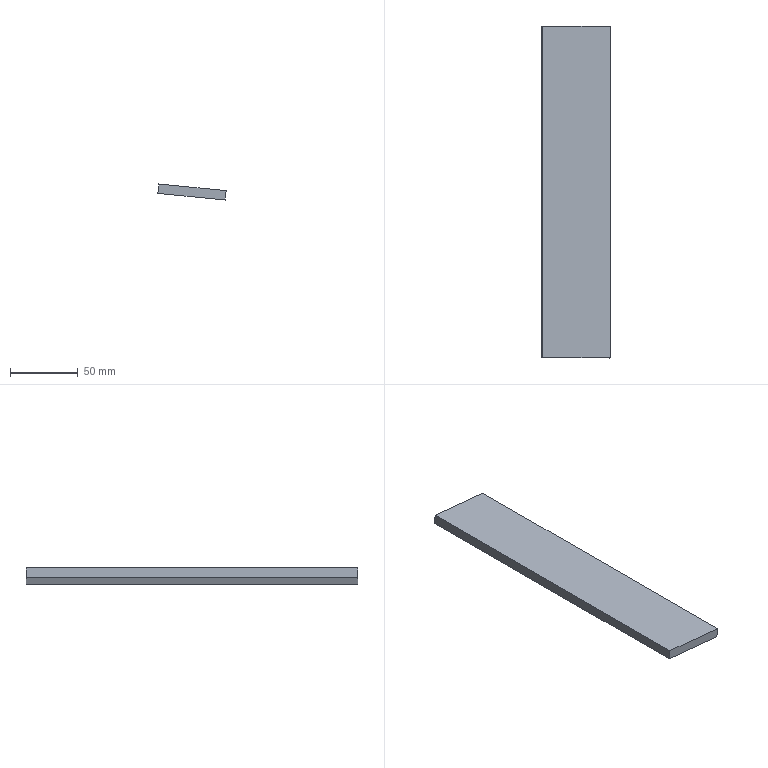Component | NX | MOVING_FRAME_BLOCK_3_2 | 1 solid | 6 faces | box 50.45 x 245 x 11.93 mm | volume 85750 mm3 | plane 6
STEP:
#1=CARTESIAN_POINT('',(0.,0.,0.));
#2=DIRECTION('',(0.,0.,1.));
#3=DIRECTION('',(1.,0.,0.));
#4=AXIS2_PLACEMENT_3D('',#1,#2,#3);
#5=CARTESIAN_POINT('',(470.025,-55.,468.347));
#6=VERTEX_POINT('',#5);
#7=CARTESIAN_POINT('',(469.329,-55.,461.382));
#8=VERTEX_POINT('',#7);
#9=CARTESIAN_POINT('',(470.025,-55.,468.347));
#10=DIRECTION('',(-0.09932,0.,-0.9951));
#11=VECTOR('',#10,1.);
#12=LINE('',#9,#11);
#13=CARTESIAN_POINT('',(470.025,190.,468.347));
#14=DIRECTION('',(-0.9951,0.,0.09932));
#15=DIRECTION('',(0.09932,0.,0.9951));
#16=AXIS2_PLACEMENT_3D('',#13,#14,#15);
#17=PLANE('',#16);
#18=CARTESIAN_POINT('',(0.,-245.));
#19=DIRECTION('',(-1.,0.));
#20=VECTOR('',#19,1.);
#21=LINE('',#18,#20);
#22=(GEOMETRIC_REPRESENTATION_CONTEXT(2)PARAMETRIC_REPRESENTATION_CONTEXT()REPRESENTATION_CONTEXT('',''));
#23=DEFINITIONAL_REPRESENTATION('',(#21),#22);
#24=PCURVE('',#17,#23);
#25=CARTESIAN_POINT('',(469.329,-55.,461.382));
#26=DIRECTION('',(0.,-1.,0.));
#27=DIRECTION('',(-0.09932,0.,-0.9951));
#28=AXIS2_PLACEMENT_3D('',#25,#26,#27);
#29=PLANE('',#28);
#30=CARTESIAN_POINT('',(-7.,-0.));
#31=DIRECTION('',(1.,0.));
#32=VECTOR('',#31,1.);
#33=LINE('',#30,#32);
#34=(GEOMETRIC_REPRESENTATION_CONTEXT(2)PARAMETRIC_REPRESENTATION_CONTEXT()REPRESENTATION_CONTEXT('',''));
#35=DEFINITIONAL_REPRESENTATION('',(#33),#34);
#36=PCURVE('',#29,#35);
#37=SURFACE_CURVE('',#12,(#24,#36),.PCURVE_S1.);
#38=EDGE_CURVE('',#6,#8,#37,.T.);
#39=ORIENTED_EDGE('',*,*,#38,.F.);
#40=CARTESIAN_POINT('',(470.025,190.,468.347));
#41=VERTEX_POINT('',#40);
#42=CARTESIAN_POINT('',(470.025,190.,468.347));
#43=DIRECTION('',(0.,-1.,0.));
#44=VECTOR('',#43,1.);
#45=LINE('',#42,#44);
#46=CARTESIAN_POINT('',(0.,0.));
#47=DIRECTION('',(0.,-1.));
#48=VECTOR('',#47,1.);
#49=LINE('',#46,#48);
#50=(GEOMETRIC_REPRESENTATION_CONTEXT(2)PARAMETRIC_REPRESENTATION_CONTEXT()REPRESENTATION_CONTEXT('',''));
#51=DEFINITIONAL_REPRESENTATION('',(#49),#50);
#52=PCURVE('',#17,#51);
#53=CARTESIAN_POINT('',(519.777,190.,463.381));
#54=DIRECTION('',(0.09932,0.,0.9951));
#55=DIRECTION('',(0.9951,0.,-0.09932));
#56=AXIS2_PLACEMENT_3D('',#53,#54,#55);
#57=PLANE('',#56);
#58=CARTESIAN_POINT('',(-50.,0.));
#59=DIRECTION('',(0.,-1.));
#60=VECTOR('',#59,1.);
#61=LINE('',#58,#60);
#62=(GEOMETRIC_REPRESENTATION_CONTEXT(2)PARAMETRIC_REPRESENTATION_CONTEXT()REPRESENTATION_CONTEXT('',''));
#63=DEFINITIONAL_REPRESENTATION('',(#61),#62);
#64=PCURVE('',#57,#63);
#65=SURFACE_CURVE('',#45,(#52,#64),.PCURVE_S1.);
#66=EDGE_CURVE('',#41,#6,#65,.T.);
#67=ORIENTED_EDGE('',*,*,#66,.F.);
#68=CARTESIAN_POINT('',(469.329,190.,461.382));
#69=VERTEX_POINT('',#68);
#70=CARTESIAN_POINT('',(470.025,190.,468.347));
#71=DIRECTION('',(-0.09932,0.,-0.9951));
#72=VECTOR('',#71,1.);
#73=LINE('',#70,#72);
#74=CARTESIAN_POINT('',(0.,0.));
#75=DIRECTION('',(-1.,0.));
#76=VECTOR('',#75,1.);
#77=LINE('',#74,#76);
#78=(GEOMETRIC_REPRESENTATION_CONTEXT(2)PARAMETRIC_REPRESENTATION_CONTEXT()REPRESENTATION_CONTEXT('',''));
#79=DEFINITIONAL_REPRESENTATION('',(#77),#78);
#80=PCURVE('',#17,#79);
#81=CARTESIAN_POINT('',(469.329,190.,461.382));
#82=DIRECTION('',(0.,-1.,0.));
#83=DIRECTION('',(-0.09932,0.,-0.9951));
#84=AXIS2_PLACEMENT_3D('',#81,#82,#83);
#85=PLANE('',#84);
#86=CARTESIAN_POINT('',(-7.,-0.));
#87=DIRECTION('',(1.,0.));
#88=VECTOR('',#87,1.);
#89=LINE('',#86,#88);
#90=(GEOMETRIC_REPRESENTATION_CONTEXT(2)PARAMETRIC_REPRESENTATION_CONTEXT()REPRESENTATION_CONTEXT('',''));
#91=DEFINITIONAL_REPRESENTATION('',(#89),#90);
#92=PCURVE('',#85,#91);
#93=SURFACE_CURVE('',#73,(#80,#92),.PCURVE_S1.);
#94=EDGE_CURVE('',#41,#69,#93,.T.);
#95=ORIENTED_EDGE('',*,*,#94,.T.);
#96=CARTESIAN_POINT('',(469.329,190.,461.382));
#97=DIRECTION('',(0.,-1.,0.));
#98=VECTOR('',#97,1.);
#99=LINE('',#96,#98);
#100=CARTESIAN_POINT('',(-7.,0.));
#101=DIRECTION('',(0.,-1.));
#102=VECTOR('',#101,1.);
#103=LINE('',#100,#102);
#104=(GEOMETRIC_REPRESENTATION_CONTEXT(2)PARAMETRIC_REPRESENTATION_CONTEXT()REPRESENTATION_CONTEXT('',''));
#105=DEFINITIONAL_REPRESENTATION('',(#103),#104);
#106=PCURVE('',#17,#105);
#107=CARTESIAN_POINT('',(469.329,190.,461.382));
#108=DIRECTION('',(-0.09932,0.,-0.9951));
#109=DIRECTION('',(-0.9951,0.,0.09932));
#110=AXIS2_PLACEMENT_3D('',#107,#108,#109);
#111=PLANE('',#110);
#112=CARTESIAN_POINT('',(0.,0.));
#113=DIRECTION('',(0.,-1.));
#114=VECTOR('',#113,1.);
#115=LINE('',#112,#114);
#116=(GEOMETRIC_REPRESENTATION_CONTEXT(2)PARAMETRIC_REPRESENTATION_CONTEXT()REPRESENTATION_CONTEXT('',''));
#117=DEFINITIONAL_REPRESENTATION('',(#115),#116);
#118=PCURVE('',#111,#117);
#119=SURFACE_CURVE('',#99,(#106,#118),.PCURVE_S1.);
#120=EDGE_CURVE('',#69,#8,#119,.T.);
#121=ORIENTED_EDGE('',*,*,#120,.T.);
#122=EDGE_LOOP('',(#39,#67,#95,#121));
#123=FACE_BOUND('',#122,.T.);
#124=ADVANCED_FACE('',(#123),#17,.T.);
#125=CARTESIAN_POINT('',(519.082,-55.,456.416));
#126=VERTEX_POINT('',#125);
#127=CARTESIAN_POINT('',(469.329,-55.,461.382));
#128=DIRECTION('',(0.9951,0.,-0.09932));
#129=VECTOR('',#128,1.);
#130=LINE('',#127,#129);
#131=CARTESIAN_POINT('',(0.,-245.));
#132=DIRECTION('',(-1.,0.));
#133=VECTOR('',#132,1.);
#134=LINE('',#131,#133);
#135=(GEOMETRIC_REPRESENTATION_CONTEXT(2)PARAMETRIC_REPRESENTATION_CONTEXT()REPRESENTATION_CONTEXT('',''));
#136=DEFINITIONAL_REPRESENTATION('',(#134),#135);
#137=PCURVE('',#111,#136);
#138=CARTESIAN_POINT('',(0.,0.));
#139=DIRECTION('',(0.,1.));
#140=VECTOR('',#139,1.);
#141=LINE('',#138,#140);
#142=(GEOMETRIC_REPRESENTATION_CONTEXT(2)PARAMETRIC_REPRESENTATION_CONTEXT()REPRESENTATION_CONTEXT('',''));
#143=DEFINITIONAL_REPRESENTATION('',(#141),#142);
#144=PCURVE('',#29,#143);
#145=SURFACE_CURVE('',#130,(#137,#144),.PCURVE_S1.);
#146=EDGE_CURVE('',#8,#126,#145,.T.);
#147=ORIENTED_EDGE('',*,*,#146,.F.);
#148=ORIENTED_EDGE('',*,*,#120,.F.);
#149=CARTESIAN_POINT('',(519.082,190.,456.416));
#150=VERTEX_POINT('',#149);
#151=CARTESIAN_POINT('',(469.329,190.,461.382));
#152=DIRECTION('',(0.9951,0.,-0.09932));
#153=VECTOR('',#152,1.);
#154=LINE('',#151,#153);
#155=CARTESIAN_POINT('',(0.,0.));
#156=DIRECTION('',(-1.,0.));
#157=VECTOR('',#156,1.);
#158=LINE('',#155,#157);
#159=(GEOMETRIC_REPRESENTATION_CONTEXT(2)PARAMETRIC_REPRESENTATION_CONTEXT()REPRESENTATION_CONTEXT('',''));
#160=DEFINITIONAL_REPRESENTATION('',(#158),#159);
#161=PCURVE('',#111,#160);
#162=CARTESIAN_POINT('',(0.,0.));
#163=DIRECTION('',(0.,1.));
#164=VECTOR('',#163,1.);
#165=LINE('',#162,#164);
#166=(GEOMETRIC_REPRESENTATION_CONTEXT(2)PARAMETRIC_REPRESENTATION_CONTEXT()REPRESENTATION_CONTEXT('',''));
#167=DEFINITIONAL_REPRESENTATION('',(#165),#166);
#168=PCURVE('',#85,#167);
#169=SURFACE_CURVE('',#154,(#161,#168),.PCURVE_S1.);
#170=EDGE_CURVE('',#69,#150,#169,.T.);
#171=ORIENTED_EDGE('',*,*,#170,.T.);
#172=CARTESIAN_POINT('',(519.082,190.,456.416));
#173=DIRECTION('',(0.,-1.,0.));
#174=VECTOR('',#173,1.);
#175=LINE('',#172,#174);
#176=CARTESIAN_POINT('',(-50.,0.));
#177=DIRECTION('',(0.,-1.));
#178=VECTOR('',#177,1.);
#179=LINE('',#176,#178);
#180=(GEOMETRIC_REPRESENTATION_CONTEXT(2)PARAMETRIC_REPRESENTATION_CONTEXT()REPRESENTATION_CONTEXT('',''));
#181=DEFINITIONAL_REPRESENTATION('',(#179),#180);
#182=PCURVE('',#111,#181);
#183=CARTESIAN_POINT('',(519.082,190.,456.416));
#184=DIRECTION('',(0.9951,0.,-0.09932));
#185=DIRECTION('',(-0.09932,0.,-0.9951));
#186=AXIS2_PLACEMENT_3D('',#183,#184,#185);
#187=PLANE('',#186);
#188=CARTESIAN_POINT('',(0.,0.));
#189=DIRECTION('',(0.,-1.));
#190=VECTOR('',#189,1.);
#191=LINE('',#188,#190);
#192=(GEOMETRIC_REPRESENTATION_CONTEXT(2)PARAMETRIC_REPRESENTATION_CONTEXT()REPRESENTATION_CONTEXT('',''));
#193=DEFINITIONAL_REPRESENTATION('',(#191),#192);
#194=PCURVE('',#187,#193);
#195=SURFACE_CURVE('',#175,(#182,#194),.PCURVE_S1.);
#196=EDGE_CURVE('',#150,#126,#195,.T.);
#197=ORIENTED_EDGE('',*,*,#196,.T.);
#198=EDGE_LOOP('',(#147,#148,#171,#197));
#199=FACE_BOUND('',#198,.T.);
#200=ADVANCED_FACE('',(#199),#111,.T.);
#201=CARTESIAN_POINT('',(519.777,-55.,463.381));
#202=VERTEX_POINT('',#201);
#203=CARTESIAN_POINT('',(519.082,-55.,456.416));
#204=DIRECTION('',(0.09932,0.,0.9951));
#205=VECTOR('',#204,1.);
#206=LINE('',#203,#205);
#207=CARTESIAN_POINT('',(0.,-245.));
#208=DIRECTION('',(-1.,0.));
#209=VECTOR('',#208,1.);
#210=LINE('',#207,#209);
#211=(GEOMETRIC_REPRESENTATION_CONTEXT(2)PARAMETRIC_REPRESENTATION_CONTEXT()REPRESENTATION_CONTEXT('',''));
#212=DEFINITIONAL_REPRESENTATION('',(#210),#211);
#213=PCURVE('',#187,#212);
#214=CARTESIAN_POINT('',(0.,50.));
#215=DIRECTION('',(-1.,0.));
#216=VECTOR('',#215,1.);
#217=LINE('',#214,#216);
#218=(GEOMETRIC_REPRESENTATION_CONTEXT(2)PARAMETRIC_REPRESENTATION_CONTEXT()REPRESENTATION_CONTEXT('',''));
#219=DEFINITIONAL_REPRESENTATION('',(#217),#218);
#220=PCURVE('',#29,#219);
#221=SURFACE_CURVE('',#206,(#213,#220),.PCURVE_S1.);
#222=EDGE_CURVE('',#126,#202,#221,.T.);
#223=ORIENTED_EDGE('',*,*,#222,.F.);
#224=ORIENTED_EDGE('',*,*,#196,.F.);
#225=CARTESIAN_POINT('',(519.777,190.,463.381));
#226=VERTEX_POINT('',#225);
#227=CARTESIAN_POINT('',(519.082,190.,456.416));
#228=DIRECTION('',(0.09932,0.,0.9951));
#229=VECTOR('',#228,1.);
#230=LINE('',#227,#229);
#231=CARTESIAN_POINT('',(0.,0.));
#232=DIRECTION('',(-1.,0.));
#233=VECTOR('',#232,1.);
#234=LINE('',#231,#233);
#235=(GEOMETRIC_REPRESENTATION_CONTEXT(2)PARAMETRIC_REPRESENTATION_CONTEXT()REPRESENTATION_CONTEXT('',''));
#236=DEFINITIONAL_REPRESENTATION('',(#234),#235);
#237=PCURVE('',#187,#236);
#238=CARTESIAN_POINT('',(0.,50.));
#239=DIRECTION('',(-1.,0.));
#240=VECTOR('',#239,1.);
#241=LINE('',#238,#240);
#242=(GEOMETRIC_REPRESENTATION_CONTEXT(2)PARAMETRIC_REPRESENTATION_CONTEXT()REPRESENTATION_CONTEXT('',''));
#243=DEFINITIONAL_REPRESENTATION('',(#241),#242);
#244=PCURVE('',#85,#243);
#245=SURFACE_CURVE('',#230,(#237,#244),.PCURVE_S1.);
#246=EDGE_CURVE('',#150,#226,#245,.T.);
#247=ORIENTED_EDGE('',*,*,#246,.T.);
#248=CARTESIAN_POINT('',(519.777,190.,463.381));
#249=DIRECTION('',(0.,-1.,0.));
#250=VECTOR('',#249,1.);
#251=LINE('',#248,#250);
#252=CARTESIAN_POINT('',(-7.,0.));
#253=DIRECTION('',(0.,-1.));
#254=VECTOR('',#253,1.);
#255=LINE('',#252,#254);
#256=(GEOMETRIC_REPRESENTATION_CONTEXT(2)PARAMETRIC_REPRESENTATION_CONTEXT()REPRESENTATION_CONTEXT('',''));
#257=DEFINITIONAL_REPRESENTATION('',(#255),#256);
#258=PCURVE('',#187,#257);
#259=CARTESIAN_POINT('',(0.,0.));
#260=DIRECTION('',(0.,-1.));
#261=VECTOR('',#260,1.);
#262=LINE('',#259,#261);
#263=(GEOMETRIC_REPRESENTATION_CONTEXT(2)PARAMETRIC_REPRESENTATION_CONTEXT()REPRESENTATION_CONTEXT('',''));
#264=DEFINITIONAL_REPRESENTATION('',(#262),#263);
#265=PCURVE('',#57,#264);
#266=SURFACE_CURVE('',#251,(#258,#265),.PCURVE_S1.);
#267=EDGE_CURVE('',#226,#202,#266,.T.);
#268=ORIENTED_EDGE('',*,*,#267,.T.);
#269=EDGE_LOOP('',(#223,#224,#247,#268));
#270=FACE_BOUND('',#269,.T.);
#271=ADVANCED_FACE('',(#270),#187,.T.);
#272=CARTESIAN_POINT('',(519.777,-55.,463.381));
#273=DIRECTION('',(-0.9951,0.,0.09932));
#274=VECTOR('',#273,1.);
#275=LINE('',#272,#274);
#276=CARTESIAN_POINT('',(0.,-245.));
#277=DIRECTION('',(-1.,0.));
#278=VECTOR('',#277,1.);
#279=LINE('',#276,#278);
#280=(GEOMETRIC_REPRESENTATION_CONTEXT(2)PARAMETRIC_REPRESENTATION_CONTEXT()REPRESENTATION_CONTEXT('',''));
#281=DEFINITIONAL_REPRESENTATION('',(#279),#280);
#282=PCURVE('',#57,#281);
#283=CARTESIAN_POINT('',(-7.,50.));
#284=DIRECTION('',(0.,-1.));
#285=VECTOR('',#284,1.);
#286=LINE('',#283,#285);
#287=(GEOMETRIC_REPRESENTATION_CONTEXT(2)PARAMETRIC_REPRESENTATION_CONTEXT()REPRESENTATION_CONTEXT('',''));
#288=DEFINITIONAL_REPRESENTATION('',(#286),#287);
#289=PCURVE('',#29,#288);
#290=SURFACE_CURVE('',#275,(#282,#289),.PCURVE_S1.);
#291=EDGE_CURVE('',#202,#6,#290,.T.);
#292=ORIENTED_EDGE('',*,*,#291,.F.);
#293=ORIENTED_EDGE('',*,*,#267,.F.);
#294=CARTESIAN_POINT('',(519.777,190.,463.381));
#295=DIRECTION('',(-0.9951,0.,0.09932));
#296=VECTOR('',#295,1.);
#297=LINE('',#294,#296);
#298=CARTESIAN_POINT('',(0.,0.));
#299=DIRECTION('',(-1.,0.));
#300=VECTOR('',#299,1.);
#301=LINE('',#298,#300);
#302=(GEOMETRIC_REPRESENTATION_CONTEXT(2)PARAMETRIC_REPRESENTATION_CONTEXT()REPRESENTATION_CONTEXT('',''));
#303=DEFINITIONAL_REPRESENTATION('',(#301),#302);
#304=PCURVE('',#57,#303);
#305=CARTESIAN_POINT('',(-7.,50.));
#306=DIRECTION('',(0.,-1.));
#307=VECTOR('',#306,1.);
#308=LINE('',#305,#307);
#309=(GEOMETRIC_REPRESENTATION_CONTEXT(2)PARAMETRIC_REPRESENTATION_CONTEXT()REPRESENTATION_CONTEXT('',''));
#310=DEFINITIONAL_REPRESENTATION('',(#308),#309);
#311=PCURVE('',#85,#310);
#312=SURFACE_CURVE('',#297,(#304,#311),.PCURVE_S1.);
#313=EDGE_CURVE('',#226,#41,#312,.T.);
#314=ORIENTED_EDGE('',*,*,#313,.T.);
#315=ORIENTED_EDGE('',*,*,#66,.T.);
#316=EDGE_LOOP('',(#292,#293,#314,#315));
#317=FACE_BOUND('',#316,.T.);
#318=ADVANCED_FACE('',(#317),#57,.T.);
#319=ORIENTED_EDGE('',*,*,#94,.F.);
#320=ORIENTED_EDGE('',*,*,#313,.F.);
#321=ORIENTED_EDGE('',*,*,#246,.F.);
#322=ORIENTED_EDGE('',*,*,#170,.F.);
#323=EDGE_LOOP('',(#319,#320,#321,#322));
#324=FACE_BOUND('',#323,.T.);
#325=ADVANCED_FACE('',(#324),#85,.F.);
#326=ORIENTED_EDGE('',*,*,#38,.T.);
#327=ORIENTED_EDGE('',*,*,#146,.T.);
#328=ORIENTED_EDGE('',*,*,#222,.T.);
#329=ORIENTED_EDGE('',*,*,#291,.T.);
#330=EDGE_LOOP('',(#326,#327,#328,#329));
#331=FACE_BOUND('',#330,.T.);
#332=ADVANCED_FACE('',(#331),#29,.T.);
#333=CLOSED_SHELL('',(#124,#200,#271,#318,#325,#332));
#334=MANIFOLD_SOLID_BREP('',#333);
#335=(LENGTH_UNIT()NAMED_UNIT(*)SI_UNIT(.MILLI.,.METRE.));
#336=UNCERTAINTY_MEASURE_WITH_UNIT(LENGTH_MEASURE(0.0000001),#335,'','');
#337=(NAMED_UNIT(*)PLANE_ANGLE_UNIT()SI_UNIT($,.RADIAN.));
#338=(NAMED_UNIT(*)SI_UNIT($,.STERADIAN.)SOLID_ANGLE_UNIT());
#339=(GEOMETRIC_REPRESENTATION_CONTEXT(3)GLOBAL_UNCERTAINTY_ASSIGNED_CONTEXT((#336))GLOBAL_UNIT_ASSIGNED_CONTEXT((#335,#337,#338))REPRESENTATION_CONTEXT('',''));
#340=ADVANCED_BREP_SHAPE_REPRESENTATION('',(#4,#334),#339);